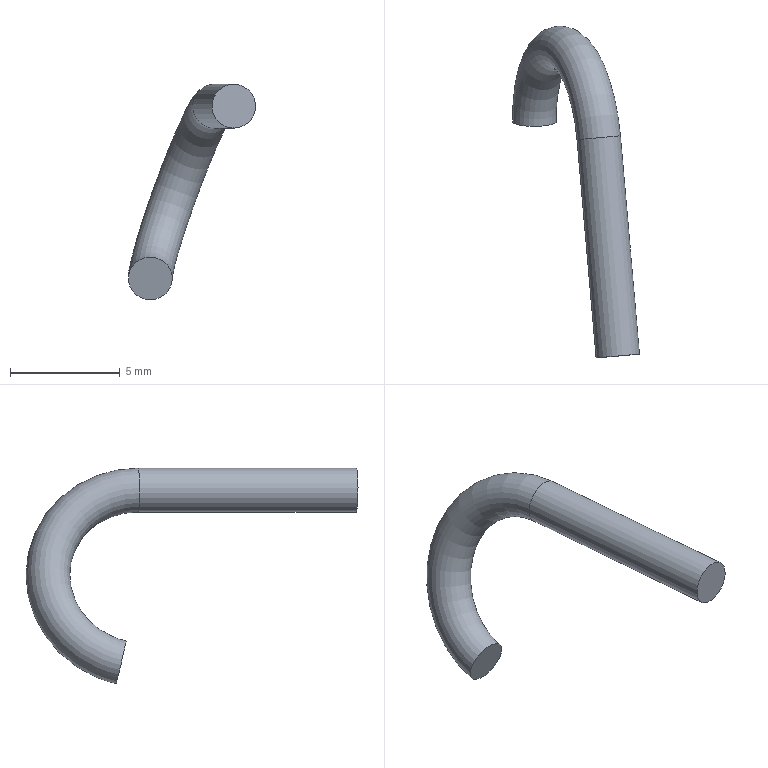Component | NX | HOOK | 1 solid | 4 faces | box 5.81 x 15.15 x 9.84 mm | volume 70 mm3 | plane 2 | torus 1 | cylinder 1 | commonest cylinder face diameters 2 x1
STEP:
#1=CARTESIAN_POINT('',(0.,0.,0.));
#2=DIRECTION('',(0.,0.,1.));
#3=DIRECTION('',(1.,0.,0.));
#4=AXIS2_PLACEMENT_3D('',#1,#2,#3);
#5=CARTESIAN_POINT('',(-1.59,58.39,-4.658));
#6=VERTEX_POINT('',#5);
#7=CARTESIAN_POINT('',(-0.6537,58.471,-5.));
#8=DIRECTION('',(-0.08716,0.9962,0.));
#9=DIRECTION('',(-0.9361,-0.0819,0.342));
#10=AXIS2_PLACEMENT_3D('',#7,#8,#9);
#11=CIRCLE('',#10,1.);
#12=CARTESIAN_POINT('',(-2.1,58.345,-8.989));
#13=DIRECTION('',(-0.9361,-0.0819,0.342));
#14=DIRECTION('',(0.08716,-0.9962,0.));
#15=AXIS2_PLACEMENT_3D('',#12,#13,#14);
#16=TOROIDAL_SURFACE('',#15,4.245,1.);
#17=CARTESIAN_POINT('',(7.854,7.854));
#18=DIRECTION('',(0.,-1.));
#19=VECTOR('',#18,1.);
#20=LINE('',#17,#19);
#21=(GEOMETRIC_REPRESENTATION_CONTEXT(2)PARAMETRIC_REPRESENTATION_CONTEXT()REPRESENTATION_CONTEXT('',''));
#22=DEFINITIONAL_REPRESENTATION('',(#20),#21);
#23=PCURVE('',#16,#22);
#24=CARTESIAN_POINT('',(-0.6537,58.471,-5.));
#25=DIRECTION('',(0.08716,-0.9962,0.));
#26=DIRECTION('',(0.9361,0.0819,-0.342));
#27=AXIS2_PLACEMENT_3D('',#24,#25,#26);
#28=CYLINDRICAL_SURFACE('',#27,1.);
#29=CARTESIAN_POINT('',(9.425,0.));
#30=DIRECTION('',(-1.,0.));
#31=VECTOR('',#30,1.);
#32=LINE('',#29,#31);
#33=(GEOMETRIC_REPRESENTATION_CONTEXT(2)PARAMETRIC_REPRESENTATION_CONTEXT()REPRESENTATION_CONTEXT('',''));
#34=DEFINITIONAL_REPRESENTATION('',(#32),#33);
#35=PCURVE('',#28,#34);
#36=SURFACE_CURVE('',#11,(#23,#35),.PCURVE_S1.);
#37=EDGE_CURVE('',#6,#6,#36,.T.);
#38=ORIENTED_EDGE('',*,*,#37,.T.);
#39=CARTESIAN_POINT('',(-4.529,59.144,-12.522));
#40=VERTEX_POINT('',#39);
#41=CARTESIAN_POINT('',(-1.59,58.39,-4.658));
#42=CARTESIAN_POINT('',(-1.724,59.924,-4.658));
#43=CARTESIAN_POINT('',(-2.076,61.439,-5.258));
#44=CARTESIAN_POINT('',(-2.618,62.627,-6.457));
#45=CARTESIAN_POINT('',(-3.263,63.187,-8.09));
#46=CARTESIAN_POINT('',(-3.872,62.949,-9.813));
#47=CARTESIAN_POINT('',(-4.316,62.014,-11.253));
#48=CARTESIAN_POINT('',(-4.535,60.645,-12.179));
#49=CARTESIAN_POINT('',(-4.529,59.144,-12.522));
#50=B_SPLINE_CURVE_WITH_KNOTS('',8,(#41,#42,#43,#44,#45,#46,#47,#48,#49),.UNSPECIFIED.,.F.,.F.,(9,9),(1.571,4.473),.PIECEWISE_BEZIER_KNOTS.);
#51=CARTESIAN_POINT('',(6.283,1.571));
#52=DIRECTION('',(1.,0.));
#53=VECTOR('',#52,1.);
#54=LINE('',#51,#53);
#55=(GEOMETRIC_REPRESENTATION_CONTEXT(2)PARAMETRIC_REPRESENTATION_CONTEXT()REPRESENTATION_CONTEXT('',''));
#56=DEFINITIONAL_REPRESENTATION('',(#54),#55);
#57=PCURVE('',#16,#56);
#58=CARTESIAN_POINT('',(6.283,7.854));
#59=DIRECTION('',(1.,0.));
#60=VECTOR('',#59,1.);
#61=LINE('',#58,#60);
#62=(GEOMETRIC_REPRESENTATION_CONTEXT(2)PARAMETRIC_REPRESENTATION_CONTEXT()REPRESENTATION_CONTEXT('',''));
#63=DEFINITIONAL_REPRESENTATION('',(#61),#62);
#64=PCURVE('',#16,#63);
#65=SEAM_CURVE('',#50,(#57,#64),.PCURVE_S1.);
#66=EDGE_CURVE('',#6,#40,#65,.T.);
#67=ORIENTED_EDGE('',*,*,#66,.T.);
#68=CARTESIAN_POINT('',(-3.593,59.226,-12.865));
#69=DIRECTION('',(0.003779,-0.9748,-0.2231));
#70=DIRECTION('',(-0.9361,-0.0819,0.342));
#71=AXIS2_PLACEMENT_3D('',#68,#69,#70);
#72=CIRCLE('',#71,1.);
#73=CARTESIAN_POINT('',(10.756,7.854));
#74=DIRECTION('',(0.,-1.));
#75=VECTOR('',#74,1.);
#76=LINE('',#73,#75);
#77=(GEOMETRIC_REPRESENTATION_CONTEXT(2)PARAMETRIC_REPRESENTATION_CONTEXT()REPRESENTATION_CONTEXT('',''));
#78=DEFINITIONAL_REPRESENTATION('',(#76),#77);
#79=PCURVE('',#16,#78);
#80=CARTESIAN_POINT('',(-3.593,59.226,-12.865));
#81=DIRECTION('',(0.003779,-0.9748,-0.2231));
#82=DIRECTION('',(-0.9361,-0.0819,0.342));
#83=AXIS2_PLACEMENT_3D('',#80,#81,#82);
#84=PLANE('',#83);
#85=CARTESIAN_POINT('',(0.,0.));
#86=DIRECTION('',(1.,-0.));
#87=AXIS2_PLACEMENT_2D('',#85,#86);
#88=CIRCLE('',#87,1.);
#89=(GEOMETRIC_REPRESENTATION_CONTEXT(2)PARAMETRIC_REPRESENTATION_CONTEXT()REPRESENTATION_CONTEXT('',''));
#90=DEFINITIONAL_REPRESENTATION('',(#88),#89);
#91=PCURVE('',#84,#90);
#92=SURFACE_CURVE('',#72,(#79,#91),.PCURVE_S1.);
#93=EDGE_CURVE('',#40,#40,#92,.T.);
#94=ORIENTED_EDGE('',*,*,#93,.F.);
#95=ORIENTED_EDGE('',*,*,#66,.F.);
#96=EDGE_LOOP('',(#38,#67,#94,#95));
#97=FACE_BOUND('',#96,.T.);
#98=ADVANCED_FACE('',(#97),#16,.T.);
#99=ORIENTED_EDGE('',*,*,#37,.F.);
#100=CARTESIAN_POINT('',(-0.7182,48.428,-4.658));
#101=VERTEX_POINT('',#100);
#102=CARTESIAN_POINT('',(-1.59,58.39,-4.658));
#103=CARTESIAN_POINT('',(-0.7182,48.428,-4.658));
#104=B_SPLINE_CURVE_WITH_KNOTS('',1,(#102,#103),.UNSPECIFIED.,.F.,.F.,(2,2),(0.,10.),.PIECEWISE_BEZIER_KNOTS.);
#105=CARTESIAN_POINT('',(9.425,0.));
#106=DIRECTION('',(0.,1.));
#107=VECTOR('',#106,1.);
#108=LINE('',#105,#107);
#109=(GEOMETRIC_REPRESENTATION_CONTEXT(2)PARAMETRIC_REPRESENTATION_CONTEXT()REPRESENTATION_CONTEXT('',''));
#110=DEFINITIONAL_REPRESENTATION('',(#108),#109);
#111=PCURVE('',#28,#110);
#112=CARTESIAN_POINT('',(3.142,0.));
#113=DIRECTION('',(0.,1.));
#114=VECTOR('',#113,1.);
#115=LINE('',#112,#114);
#116=(GEOMETRIC_REPRESENTATION_CONTEXT(2)PARAMETRIC_REPRESENTATION_CONTEXT()REPRESENTATION_CONTEXT('',''));
#117=DEFINITIONAL_REPRESENTATION('',(#115),#116);
#118=PCURVE('',#28,#117);
#119=SEAM_CURVE('',#104,(#111,#118),.PCURVE_S1.);
#120=EDGE_CURVE('',#6,#101,#119,.T.);
#121=ORIENTED_EDGE('',*,*,#120,.T.);
#122=CARTESIAN_POINT('',(0.2179,48.51,-5.));
#123=DIRECTION('',(-0.08716,0.9962,0.));
#124=DIRECTION('',(-0.9361,-0.0819,0.342));
#125=AXIS2_PLACEMENT_3D('',#122,#123,#124);
#126=CIRCLE('',#125,1.);
#127=CARTESIAN_POINT('',(9.425,10.));
#128=DIRECTION('',(-1.,0.));
#129=VECTOR('',#128,1.);
#130=LINE('',#127,#129);
#131=(GEOMETRIC_REPRESENTATION_CONTEXT(2)PARAMETRIC_REPRESENTATION_CONTEXT()REPRESENTATION_CONTEXT('',''));
#132=DEFINITIONAL_REPRESENTATION('',(#130),#131);
#133=PCURVE('',#28,#132);
#134=CARTESIAN_POINT('',(0.2179,48.51,-5.));
#135=DIRECTION('',(-0.08716,0.9962,0.));
#136=DIRECTION('',(-0.9361,-0.0819,0.342));
#137=AXIS2_PLACEMENT_3D('',#134,#135,#136);
#138=PLANE('',#137);
#139=CARTESIAN_POINT('',(0.,0.));
#140=DIRECTION('',(1.,-0.));
#141=AXIS2_PLACEMENT_2D('',#139,#140);
#142=CIRCLE('',#141,1.);
#143=(GEOMETRIC_REPRESENTATION_CONTEXT(2)PARAMETRIC_REPRESENTATION_CONTEXT()REPRESENTATION_CONTEXT('',''));
#144=DEFINITIONAL_REPRESENTATION('',(#142),#143);
#145=PCURVE('',#138,#144);
#146=SURFACE_CURVE('',#126,(#133,#145),.PCURVE_S1.);
#147=EDGE_CURVE('',#101,#101,#146,.T.);
#148=ORIENTED_EDGE('',*,*,#147,.T.);
#149=ORIENTED_EDGE('',*,*,#120,.F.);
#150=EDGE_LOOP('',(#99,#121,#148,#149));
#151=FACE_BOUND('',#150,.T.);
#152=ADVANCED_FACE('',(#151),#28,.T.);
#153=ORIENTED_EDGE('',*,*,#93,.T.);
#154=EDGE_LOOP('',(#153));
#155=FACE_BOUND('',#154,.T.);
#156=ADVANCED_FACE('',(#155),#84,.T.);
#157=ORIENTED_EDGE('',*,*,#147,.F.);
#158=EDGE_LOOP('',(#157));
#159=FACE_BOUND('',#158,.T.);
#160=ADVANCED_FACE('',(#159),#138,.F.);
#161=CLOSED_SHELL('',(#98,#152,#156,#160));
#162=MANIFOLD_SOLID_BREP('',#161);
#163=(LENGTH_UNIT()NAMED_UNIT(*)SI_UNIT(.MILLI.,.METRE.));
#164=UNCERTAINTY_MEASURE_WITH_UNIT(LENGTH_MEASURE(0.00001),#163,'','');
#165=(NAMED_UNIT(*)PLANE_ANGLE_UNIT()SI_UNIT($,.RADIAN.));
#166=(NAMED_UNIT(*)SI_UNIT($,.STERADIAN.)SOLID_ANGLE_UNIT());
#167=(GEOMETRIC_REPRESENTATION_CONTEXT(3)GLOBAL_UNCERTAINTY_ASSIGNED_CONTEXT((#164))GLOBAL_UNIT_ASSIGNED_CONTEXT((#163,#165,#166))REPRESENTATION_CONTEXT('',''));
#168=ADVANCED_BREP_SHAPE_REPRESENTATION('',(#4,#162),#167);